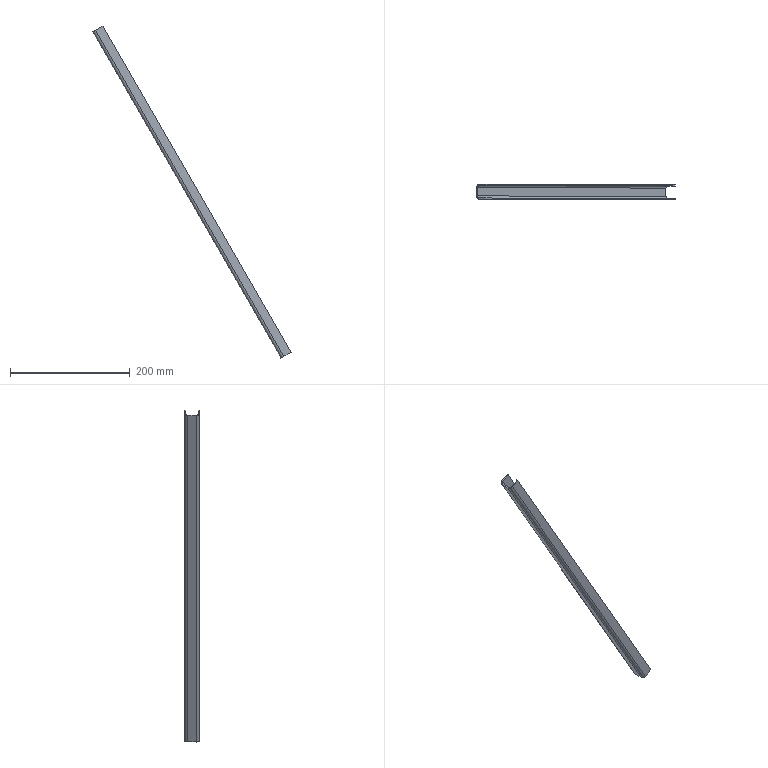Component | SolidWorks | FrontDoorAssembly-1_DoorUpperAndLowerReinforcementBar-2 | 1 solid | 22 faces | box 332.32 x 25 x 555.6 mm | volume 71993 mm3 | plane 18 | cylinder 4 | commonest cylinder face diameters 11 x2 7 x2 | material Malleable Cast Iron
STEP:
#1=COLOUR_RGB('',0.7922,0.8196,0.9333);
#2=FILL_AREA_STYLE_COLOUR('',#1);
#3=FILL_AREA_STYLE('',(#2));
#4=SURFACE_STYLE_FILL_AREA(#3);
#5=SURFACE_SIDE_STYLE('',(#4));
#6=SURFACE_STYLE_USAGE(.BOTH.,#5);
#7=PRESENTATION_STYLE_ASSIGNMENT((#6));
#8=CARTESIAN_POINT('',(10.14,-0.5527,18.399));
#9=VERTEX_POINT('',#8);
#10=CARTESIAN_POINT('',(10.208,-0.5527,18.438));
#11=VERTEX_POINT('',#10);
#12=CARTESIAN_POINT('',(10.14,-0.5527,18.399));
#13=DIRECTION('',(0.866,0.,0.5));
#14=VECTOR('',#13,39.37);
#15=LINE('',#12,#14);
#16=EDGE_CURVE('',#9,#11,#15,.T.);
#17=ORIENTED_EDGE('',*,*,#16,.F.);
#18=CARTESIAN_POINT('',(10.327,-0.3362,18.507));
#19=VERTEX_POINT('',#18);
#20=CARTESIAN_POINT('',(10.327,-0.5527,18.507));
#21=DIRECTION('',(-0.5,-0.,0.866));
#22=DIRECTION('',(0.866,0.,0.5));
#23=AXIS2_PLACEMENT_3D('',#20,#21,#22);
#24=CIRCLE('',#23,0.2165);
#25=EDGE_CURVE('',#19,#9,#24,.T.);
#26=ORIENTED_EDGE('',*,*,#25,.F.);
#27=CARTESIAN_POINT('',(10.327,-0.4149,18.507));
#28=VERTEX_POINT('',#27);
#29=CARTESIAN_POINT('',(10.327,-0.4149,18.507));
#30=DIRECTION('',(-0.,1.,0.));
#31=VECTOR('',#30,39.37);
#32=LINE('',#29,#31);
#33=EDGE_CURVE('',#28,#19,#32,.T.);
#34=ORIENTED_EDGE('',*,*,#33,.F.);
#35=CARTESIAN_POINT('',(10.327,-0.5527,18.507));
#36=DIRECTION('',(-0.5,-0.,0.866));
#37=DIRECTION('',(0.,-1.,0.));
#38=AXIS2_PLACEMENT_3D('',#35,#36,#37);
#39=CIRCLE('',#38,0.1378);
#40=EDGE_CURVE('',#28,#11,#39,.T.);
#41=ORIENTED_EDGE('',*,*,#40,.T.);
#42=EDGE_LOOP('',(#17,#26,#34,#41));
#43=FACE_OUTER_BOUND('',#42,.T.);
#44=CARTESIAN_POINT('',(10.14,-0.5527,18.399));
#45=DIRECTION('',(0.5,0.,-0.866));
#46=DIRECTION('',(0.866,0.,0.5));
#47=AXIS2_PLACEMENT_3D('',#44,#45,#46);
#48=PLANE('',#47);
#49=ADVANCED_FACE('',(#43),#48,.T.);
#50=CARTESIAN_POINT('',(10.14,-1.104,18.399));
#51=VERTEX_POINT('',#50);
#52=CARTESIAN_POINT('',(10.14,-0.3362,18.399));
#53=DIRECTION('',(0.,-1.,-0.));
#54=VECTOR('',#53,39.37);
#55=LINE('',#52,#54);
#56=EDGE_CURVE('',#9,#51,#55,.T.);
#57=ORIENTED_EDGE('',*,*,#56,.F.);
#58=ORIENTED_EDGE('',*,*,#16,.T.);
#59=CARTESIAN_POINT('',(10.208,-1.104,18.438));
#60=VERTEX_POINT('',#59);
#61=CARTESIAN_POINT('',(10.208,-0.3362,18.438));
#62=DIRECTION('',(0.,-1.,-0.));
#63=VECTOR('',#62,39.37);
#64=LINE('',#61,#63);
#65=EDGE_CURVE('',#11,#60,#64,.T.);
#66=ORIENTED_EDGE('',*,*,#65,.T.);
#67=CARTESIAN_POINT('',(10.208,-1.104,18.438));
#68=DIRECTION('',(-0.866,-0.,-0.5));
#69=VECTOR('',#68,39.37);
#70=LINE('',#67,#69);
#71=EDGE_CURVE('',#60,#51,#70,.T.);
#72=ORIENTED_EDGE('',*,*,#71,.T.);
#73=EDGE_LOOP('',(#57,#58,#66,#72));
#74=FACE_OUTER_BOUND('',#73,.T.);
#75=CARTESIAN_POINT('',(10.327,-0.4149,18.507));
#76=DIRECTION('',(0.5,0.,-0.866));
#77=DIRECTION('',(0.866,0.,0.5));
#78=AXIS2_PLACEMENT_3D('',#75,#76,#77);
#79=PLANE('',#78);
#80=ADVANCED_FACE('',(#74),#79,.T.);
#81=CARTESIAN_POINT('',(-2.074,-0.3362,39.987));
#82=VERTEX_POINT('',#81);
#83=CARTESIAN_POINT('',(-2.074,-0.4149,39.987));
#84=VERTEX_POINT('',#83);
#85=CARTESIAN_POINT('',(-2.074,-0.3362,39.987));
#86=DIRECTION('',(0.,-1.,-0.));
#87=VECTOR('',#86,39.37);
#88=LINE('',#85,#87);
#89=EDGE_CURVE('',#82,#84,#88,.T.);
#90=ORIENTED_EDGE('',*,*,#89,.F.);
#91=CARTESIAN_POINT('',(-2.262,-0.5527,39.879));
#92=VERTEX_POINT('',#91);
#93=CARTESIAN_POINT('',(-2.074,-0.5527,39.987));
#94=DIRECTION('',(-0.5,-0.,0.866));
#95=DIRECTION('',(0.866,-0.,0.5));
#96=AXIS2_PLACEMENT_3D('',#93,#94,#95);
#97=CIRCLE('',#96,0.2165);
#98=EDGE_CURVE('',#82,#92,#97,.T.);
#99=ORIENTED_EDGE('',*,*,#98,.T.);
#100=CARTESIAN_POINT('',(-2.193,-0.5527,39.918));
#101=VERTEX_POINT('',#100);
#102=CARTESIAN_POINT('',(-2.193,-0.5527,39.918));
#103=DIRECTION('',(-0.866,-0.,-0.5));
#104=VECTOR('',#103,39.37);
#105=LINE('',#102,#104);
#106=EDGE_CURVE('',#101,#92,#105,.T.);
#107=ORIENTED_EDGE('',*,*,#106,.F.);
#108=CARTESIAN_POINT('',(-2.074,-0.5527,39.987));
#109=DIRECTION('',(-0.5,-0.,0.866));
#110=DIRECTION('',(-0.,-1.,-0.));
#111=AXIS2_PLACEMENT_3D('',#108,#109,#110);
#112=CIRCLE('',#111,0.1378);
#113=EDGE_CURVE('',#84,#101,#112,.T.);
#114=ORIENTED_EDGE('',*,*,#113,.F.);
#115=EDGE_LOOP('',(#90,#99,#107,#114));
#116=FACE_OUTER_BOUND('',#115,.T.);
#117=CARTESIAN_POINT('',(-2.074,-0.3362,39.987));
#118=DIRECTION('',(-0.5,-0.,0.866));
#119=DIRECTION('',(-0.866,-0.,-0.5));
#120=AXIS2_PLACEMENT_3D('',#117,#118,#119);
#121=PLANE('',#120);
#122=ADVANCED_FACE('',(#116),#121,.T.);
#123=CARTESIAN_POINT('',(-1.58,-0.3362,40.273));
#124=VERTEX_POINT('',#123);
#125=CARTESIAN_POINT('',(-1.58,-0.3362,40.273));
#126=DIRECTION('',(-0.866,-0.,-0.5));
#127=VECTOR('',#126,39.37);
#128=LINE('',#125,#127);
#129=EDGE_CURVE('',#124,#82,#128,.T.);
#130=ORIENTED_EDGE('',*,*,#129,.T.);
#131=ORIENTED_EDGE('',*,*,#89,.T.);
#132=CARTESIAN_POINT('',(-1.58,-0.4149,40.273));
#133=VERTEX_POINT('',#132);
#134=CARTESIAN_POINT('',(-1.58,-0.4149,40.273));
#135=DIRECTION('',(-0.866,-0.,-0.5));
#136=VECTOR('',#135,39.37);
#137=LINE('',#134,#136);
#138=EDGE_CURVE('',#133,#84,#137,.T.);
#139=ORIENTED_EDGE('',*,*,#138,.F.);
#140=CARTESIAN_POINT('',(-1.58,-0.4149,40.273));
#141=DIRECTION('',(-0.,1.,0.));
#142=VECTOR('',#141,39.37);
#143=LINE('',#140,#142);
#144=EDGE_CURVE('',#133,#124,#143,.T.);
#145=ORIENTED_EDGE('',*,*,#144,.T.);
#146=EDGE_LOOP('',(#130,#131,#139,#145));
#147=FACE_OUTER_BOUND('',#146,.T.);
#148=CARTESIAN_POINT('',(-2.193,-0.5527,39.918));
#149=DIRECTION('',(-0.5,-0.,0.866));
#150=DIRECTION('',(-0.866,-0.,-0.5));
#151=AXIS2_PLACEMENT_3D('',#148,#149,#150);
#152=PLANE('',#151);
#153=ADVANCED_FACE('',(#147),#152,.T.);
#154=CARTESIAN_POINT('',(10.327,-1.32,18.507));
#155=VERTEX_POINT('',#154);
#156=CARTESIAN_POINT('',(10.327,-1.242,18.507));
#157=VERTEX_POINT('',#156);
#158=CARTESIAN_POINT('',(10.327,-1.32,18.507));
#159=DIRECTION('',(-0.,1.,0.));
#160=VECTOR('',#159,39.37);
#161=LINE('',#158,#160);
#162=EDGE_CURVE('',#155,#157,#161,.T.);
#163=ORIENTED_EDGE('',*,*,#162,.F.);
#164=CARTESIAN_POINT('',(10.327,-1.104,18.507));
#165=DIRECTION('',(-0.5,-0.,0.866));
#166=DIRECTION('',(0.866,0.,0.5));
#167=AXIS2_PLACEMENT_3D('',#164,#165,#166);
#168=CIRCLE('',#167,0.2165);
#169=EDGE_CURVE('',#51,#155,#168,.T.);
#170=ORIENTED_EDGE('',*,*,#169,.F.);
#171=ORIENTED_EDGE('',*,*,#71,.F.);
#172=CARTESIAN_POINT('',(10.327,-1.104,18.507));
#173=DIRECTION('',(-0.5,-0.,0.866));
#174=DIRECTION('',(-0.,-1.,-0.));
#175=AXIS2_PLACEMENT_3D('',#172,#173,#174);
#176=CIRCLE('',#175,0.1378);
#177=EDGE_CURVE('',#60,#157,#176,.T.);
#178=ORIENTED_EDGE('',*,*,#177,.T.);
#179=EDGE_LOOP('',(#163,#170,#171,#178));
#180=FACE_OUTER_BOUND('',#179,.T.);
#181=CARTESIAN_POINT('',(10.327,-1.32,18.507));
#182=DIRECTION('',(0.5,0.,-0.866));
#183=DIRECTION('',(0.866,0.,0.5));
#184=AXIS2_PLACEMENT_3D('',#181,#182,#183);
#185=PLANE('',#184);
#186=ADVANCED_FACE('',(#180),#185,.T.);
#187=CARTESIAN_POINT('',(10.822,-1.32,18.793));
#188=VERTEX_POINT('',#187);
#189=CARTESIAN_POINT('',(10.14,-1.32,18.399));
#190=DIRECTION('',(0.866,0.,0.5));
#191=VECTOR('',#190,39.37);
#192=LINE('',#189,#191);
#193=EDGE_CURVE('',#155,#188,#192,.T.);
#194=ORIENTED_EDGE('',*,*,#193,.F.);
#195=ORIENTED_EDGE('',*,*,#162,.T.);
#196=CARTESIAN_POINT('',(10.822,-1.242,18.793));
#197=VERTEX_POINT('',#196);
#198=CARTESIAN_POINT('',(10.14,-1.242,18.399));
#199=DIRECTION('',(0.866,0.,0.5));
#200=VECTOR('',#199,39.37);
#201=LINE('',#198,#200);
#202=EDGE_CURVE('',#157,#197,#201,.T.);
#203=ORIENTED_EDGE('',*,*,#202,.T.);
#204=CARTESIAN_POINT('',(10.822,-1.32,18.793));
#205=DIRECTION('',(-0.,1.,0.));
#206=VECTOR('',#205,39.37);
#207=LINE('',#204,#206);
#208=EDGE_CURVE('',#188,#197,#207,.T.);
#209=ORIENTED_EDGE('',*,*,#208,.F.);
#210=EDGE_LOOP('',(#194,#195,#203,#209));
#211=FACE_OUTER_BOUND('',#210,.T.);
#212=CARTESIAN_POINT('',(10.208,-1.104,18.438));
#213=DIRECTION('',(0.5,0.,-0.866));
#214=DIRECTION('',(0.866,0.,0.5));
#215=AXIS2_PLACEMENT_3D('',#212,#213,#214);
#216=PLANE('',#215);
#217=ADVANCED_FACE('',(#211),#216,.T.);
#218=CARTESIAN_POINT('',(-2.262,-1.104,39.879));
#219=VERTEX_POINT('',#218);
#220=CARTESIAN_POINT('',(-2.193,-1.104,39.918));
#221=VERTEX_POINT('',#220);
#222=CARTESIAN_POINT('',(-2.262,-1.104,39.879));
#223=DIRECTION('',(0.866,0.,0.5));
#224=VECTOR('',#223,39.37);
#225=LINE('',#222,#224);
#226=EDGE_CURVE('',#219,#221,#225,.T.);
#227=ORIENTED_EDGE('',*,*,#226,.F.);
#228=CARTESIAN_POINT('',(-2.074,-1.32,39.987));
#229=VERTEX_POINT('',#228);
#230=CARTESIAN_POINT('',(-2.074,-1.104,39.987));
#231=DIRECTION('',(-0.5,-0.,0.866));
#232=DIRECTION('',(0.866,-0.,0.5));
#233=AXIS2_PLACEMENT_3D('',#230,#231,#232);
#234=CIRCLE('',#233,0.2165);
#235=EDGE_CURVE('',#219,#229,#234,.T.);
#236=ORIENTED_EDGE('',*,*,#235,.T.);
#237=CARTESIAN_POINT('',(-2.074,-1.242,39.987));
#238=VERTEX_POINT('',#237);
#239=CARTESIAN_POINT('',(-2.074,-1.242,39.987));
#240=DIRECTION('',(0.,-1.,-0.));
#241=VECTOR('',#240,39.37);
#242=LINE('',#239,#241);
#243=EDGE_CURVE('',#238,#229,#242,.T.);
#244=ORIENTED_EDGE('',*,*,#243,.F.);
#245=CARTESIAN_POINT('',(-2.074,-1.104,39.987));
#246=DIRECTION('',(-0.5,-0.,0.866));
#247=DIRECTION('',(-0.,-1.,0.));
#248=AXIS2_PLACEMENT_3D('',#245,#246,#247);
#249=CIRCLE('',#248,0.1378);
#250=EDGE_CURVE('',#221,#238,#249,.T.);
#251=ORIENTED_EDGE('',*,*,#250,.F.);
#252=EDGE_LOOP('',(#227,#236,#244,#251));
#253=FACE_OUTER_BOUND('',#252,.T.);
#254=CARTESIAN_POINT('',(-2.262,-1.104,39.879));
#255=DIRECTION('',(-0.5,-0.,0.866));
#256=DIRECTION('',(-0.866,-0.,-0.5));
#257=AXIS2_PLACEMENT_3D('',#254,#255,#256);
#258=PLANE('',#257);
#259=ADVANCED_FACE('',(#253),#258,.T.);
#260=CARTESIAN_POINT('',(-2.262,-0.3362,39.879));
#261=DIRECTION('',(0.,-1.,-0.));
#262=VECTOR('',#261,39.37);
#263=LINE('',#260,#262);
#264=EDGE_CURVE('',#92,#219,#263,.T.);
#265=ORIENTED_EDGE('',*,*,#264,.T.);
#266=ORIENTED_EDGE('',*,*,#226,.T.);
#267=CARTESIAN_POINT('',(-2.193,-0.3362,39.918));
#268=DIRECTION('',(0.,-1.,-0.));
#269=VECTOR('',#268,39.37);
#270=LINE('',#267,#269);
#271=EDGE_CURVE('',#101,#221,#270,.T.);
#272=ORIENTED_EDGE('',*,*,#271,.F.);
#273=ORIENTED_EDGE('',*,*,#106,.T.);
#274=EDGE_LOOP('',(#265,#266,#272,#273));
#275=FACE_OUTER_BOUND('',#274,.T.);
#276=CARTESIAN_POINT('',(-2.074,-1.242,39.987));
#277=DIRECTION('',(-0.5,-0.,0.866));
#278=DIRECTION('',(-0.866,-0.,-0.5));
#279=AXIS2_PLACEMENT_3D('',#276,#277,#278);
#280=PLANE('',#279);
#281=ADVANCED_FACE('',(#275),#280,.T.);
#282=CARTESIAN_POINT('',(-1.58,-1.242,40.273));
#283=VERTEX_POINT('',#282);
#284=CARTESIAN_POINT('',(-2.262,-1.242,39.879));
#285=DIRECTION('',(0.866,0.,0.5));
#286=VECTOR('',#285,39.37);
#287=LINE('',#284,#286);
#288=EDGE_CURVE('',#238,#283,#287,.T.);
#289=ORIENTED_EDGE('',*,*,#288,.T.);
#290=CARTESIAN_POINT('',(10.822,-1.242,18.793));
#291=DIRECTION('',(-0.5,-0.,0.866));
#292=VECTOR('',#291,39.37);
#293=LINE('',#290,#292);
#294=EDGE_CURVE('',#197,#283,#293,.T.);
#295=ORIENTED_EDGE('',*,*,#294,.F.);
#296=ORIENTED_EDGE('',*,*,#202,.F.);
#297=CARTESIAN_POINT('',(10.327,-1.242,18.507));
#298=DIRECTION('',(-0.5,-0.,0.866));
#299=VECTOR('',#298,39.37);
#300=LINE('',#297,#299);
#301=EDGE_CURVE('',#157,#238,#300,.T.);
#302=ORIENTED_EDGE('',*,*,#301,.T.);
#303=EDGE_LOOP('',(#289,#295,#296,#302));
#304=FACE_OUTER_BOUND('',#303,.T.);
#305=CARTESIAN_POINT('',(10.14,-1.242,18.399));
#306=DIRECTION('',(0.,-1.,-0.));
#307=DIRECTION('',(-0.866,-0.,-0.5));
#308=AXIS2_PLACEMENT_3D('',#305,#306,#307);
#309=PLANE('',#308);
#310=ADVANCED_FACE('',(#304),#309,.F.);
#311=CARTESIAN_POINT('',(-1.58,-1.32,40.273));
#312=VERTEX_POINT('',#311);
#313=CARTESIAN_POINT('',(-1.58,-1.32,40.273));
#314=DIRECTION('',(-0.,1.,0.));
#315=VECTOR('',#314,39.37);
#316=LINE('',#313,#315);
#317=EDGE_CURVE('',#312,#283,#316,.T.);
#318=ORIENTED_EDGE('',*,*,#317,.F.);
#319=CARTESIAN_POINT('',(10.822,-1.32,18.793));
#320=DIRECTION('',(-0.5,-0.,0.866));
#321=VECTOR('',#320,39.37);
#322=LINE('',#319,#321);
#323=EDGE_CURVE('',#188,#312,#322,.T.);
#324=ORIENTED_EDGE('',*,*,#323,.F.);
#325=ORIENTED_EDGE('',*,*,#208,.T.);
#326=ORIENTED_EDGE('',*,*,#294,.T.);
#327=EDGE_LOOP('',(#318,#324,#325,#326));
#328=FACE_OUTER_BOUND('',#327,.T.);
#329=CARTESIAN_POINT('',(10.822,-1.32,18.793));
#330=DIRECTION('',(0.866,0.,0.5));
#331=DIRECTION('',(0.,-1.,-0.));
#332=AXIS2_PLACEMENT_3D('',#329,#330,#331);
#333=PLANE('',#332);
#334=ADVANCED_FACE('',(#328),#333,.T.);
#335=CARTESIAN_POINT('',(-2.262,-1.32,39.879));
#336=DIRECTION('',(0.866,0.,0.5));
#337=VECTOR('',#336,39.37);
#338=LINE('',#335,#337);
#339=EDGE_CURVE('',#229,#312,#338,.T.);
#340=ORIENTED_EDGE('',*,*,#339,.F.);
#341=CARTESIAN_POINT('',(10.327,-1.32,18.507));
#342=DIRECTION('',(-0.5,-0.,0.866));
#343=VECTOR('',#342,39.37);
#344=LINE('',#341,#343);
#345=EDGE_CURVE('',#155,#229,#344,.T.);
#346=ORIENTED_EDGE('',*,*,#345,.F.);
#347=ORIENTED_EDGE('',*,*,#193,.T.);
#348=ORIENTED_EDGE('',*,*,#323,.T.);
#349=EDGE_LOOP('',(#340,#346,#347,#348));
#350=FACE_OUTER_BOUND('',#349,.T.);
#351=CARTESIAN_POINT('',(10.14,-1.32,18.399));
#352=DIRECTION('',(0.,-1.,-0.));
#353=DIRECTION('',(-0.866,-0.,-0.5));
#354=AXIS2_PLACEMENT_3D('',#351,#352,#353);
#355=PLANE('',#354);
#356=ADVANCED_FACE('',(#350),#355,.T.);
#357=ORIENTED_EDGE('',*,*,#235,.F.);
#358=CARTESIAN_POINT('',(10.14,-1.104,18.399));
#359=DIRECTION('',(-0.5,-0.,0.866));
#360=VECTOR('',#359,39.37);
#361=LINE('',#358,#360);
#362=EDGE_CURVE('',#51,#219,#361,.T.);
#363=ORIENTED_EDGE('',*,*,#362,.F.);
#364=ORIENTED_EDGE('',*,*,#169,.T.);
#365=ORIENTED_EDGE('',*,*,#345,.T.);
#366=EDGE_LOOP('',(#357,#363,#364,#365));
#367=FACE_OUTER_BOUND('',#366,.T.);
#368=CARTESIAN_POINT('',(10.327,-1.104,18.507));
#369=DIRECTION('',(-0.5,-0.,0.866));
#370=DIRECTION('',(-0.866,-0.,-0.5));
#371=AXIS2_PLACEMENT_3D('',#368,#369,#370);
#372=CYLINDRICAL_SURFACE('',#371,0.2165);
#373=ADVANCED_FACE('',(#367),#372,.T.);
#374=ORIENTED_EDGE('',*,*,#264,.F.);
#375=CARTESIAN_POINT('',(10.14,-0.5527,18.399));
#376=DIRECTION('',(-0.5,-0.,0.866));
#377=VECTOR('',#376,39.37);
#378=LINE('',#375,#377);
#379=EDGE_CURVE('',#9,#92,#378,.T.);
#380=ORIENTED_EDGE('',*,*,#379,.F.);
#381=ORIENTED_EDGE('',*,*,#56,.T.);
#382=ORIENTED_EDGE('',*,*,#362,.T.);
#383=EDGE_LOOP('',(#374,#380,#381,#382));
#384=FACE_OUTER_BOUND('',#383,.T.);
#385=CARTESIAN_POINT('',(10.14,-0.3362,18.399));
#386=DIRECTION('',(-0.866,-0.,-0.5));
#387=DIRECTION('',(-0.,1.,0.));
#388=AXIS2_PLACEMENT_3D('',#385,#386,#387);
#389=PLANE('',#388);
#390=ADVANCED_FACE('',(#384),#389,.T.);
#391=ORIENTED_EDGE('',*,*,#98,.F.);
#392=CARTESIAN_POINT('',(10.327,-0.3362,18.507));
#393=DIRECTION('',(-0.5,-0.,0.866));
#394=VECTOR('',#393,39.37);
#395=LINE('',#392,#394);
#396=EDGE_CURVE('',#19,#82,#395,.T.);
#397=ORIENTED_EDGE('',*,*,#396,.F.);
#398=ORIENTED_EDGE('',*,*,#25,.T.);
#399=ORIENTED_EDGE('',*,*,#379,.T.);
#400=EDGE_LOOP('',(#391,#397,#398,#399));
#401=FACE_OUTER_BOUND('',#400,.T.);
#402=CARTESIAN_POINT('',(10.327,-0.5527,18.507));
#403=DIRECTION('',(-0.5,-0.,0.866));
#404=DIRECTION('',(-0.866,-0.,-0.5));
#405=AXIS2_PLACEMENT_3D('',#402,#403,#404);
#406=CYLINDRICAL_SURFACE('',#405,0.2165);
#407=ADVANCED_FACE('',(#401),#406,.T.);
#408=ORIENTED_EDGE('',*,*,#129,.F.);
#409=CARTESIAN_POINT('',(10.822,-0.3362,18.793));
#410=VERTEX_POINT('',#409);
#411=CARTESIAN_POINT('',(10.822,-0.3362,18.793));
#412=DIRECTION('',(-0.5,-0.,0.866));
#413=VECTOR('',#412,39.37);
#414=LINE('',#411,#413);
#415=EDGE_CURVE('',#410,#124,#414,.T.);
#416=ORIENTED_EDGE('',*,*,#415,.F.);
#417=CARTESIAN_POINT('',(10.822,-0.3362,18.793));
#418=DIRECTION('',(-0.866,-0.,-0.5));
#419=VECTOR('',#418,39.37);
#420=LINE('',#417,#419);
#421=EDGE_CURVE('',#410,#19,#420,.T.);
#422=ORIENTED_EDGE('',*,*,#421,.T.);
#423=ORIENTED_EDGE('',*,*,#396,.T.);
#424=EDGE_LOOP('',(#408,#416,#422,#423));
#425=FACE_OUTER_BOUND('',#424,.T.);
#426=CARTESIAN_POINT('',(10.822,-0.3362,18.793));
#427=DIRECTION('',(-0.,1.,0.));
#428=DIRECTION('',(0.866,0.,0.5));
#429=AXIS2_PLACEMENT_3D('',#426,#427,#428);
#430=PLANE('',#429);
#431=ADVANCED_FACE('',(#425),#430,.T.);
#432=ORIENTED_EDGE('',*,*,#144,.F.);
#433=CARTESIAN_POINT('',(10.822,-0.4149,18.793));
#434=VERTEX_POINT('',#433);
#435=CARTESIAN_POINT('',(10.822,-0.4149,18.793));
#436=DIRECTION('',(-0.5,-0.,0.866));
#437=VECTOR('',#436,39.37);
#438=LINE('',#435,#437);
#439=EDGE_CURVE('',#434,#133,#438,.T.);
#440=ORIENTED_EDGE('',*,*,#439,.F.);
#441=CARTESIAN_POINT('',(10.822,-0.4149,18.793));
#442=DIRECTION('',(-0.,1.,0.));
#443=VECTOR('',#442,39.37);
#444=LINE('',#441,#443);
#445=EDGE_CURVE('',#434,#410,#444,.T.);
#446=ORIENTED_EDGE('',*,*,#445,.T.);
#447=ORIENTED_EDGE('',*,*,#415,.T.);
#448=EDGE_LOOP('',(#432,#440,#446,#447));
#449=FACE_OUTER_BOUND('',#448,.T.);
#450=CARTESIAN_POINT('',(10.822,-0.4149,18.793));
#451=DIRECTION('',(0.866,0.,0.5));
#452=DIRECTION('',(0.,-1.,-0.));
#453=AXIS2_PLACEMENT_3D('',#450,#451,#452);
#454=PLANE('',#453);
#455=ADVANCED_FACE('',(#449),#454,.T.);
#456=ORIENTED_EDGE('',*,*,#138,.T.);
#457=CARTESIAN_POINT('',(10.327,-0.4149,18.507));
#458=DIRECTION('',(-0.5,-0.,0.866));
#459=VECTOR('',#458,39.37);
#460=LINE('',#457,#459);
#461=EDGE_CURVE('',#28,#84,#460,.T.);
#462=ORIENTED_EDGE('',*,*,#461,.F.);
#463=CARTESIAN_POINT('',(10.822,-0.4149,18.793));
#464=DIRECTION('',(-0.866,-0.,-0.5));
#465=VECTOR('',#464,39.37);
#466=LINE('',#463,#465);
#467=EDGE_CURVE('',#434,#28,#466,.T.);
#468=ORIENTED_EDGE('',*,*,#467,.F.);
#469=ORIENTED_EDGE('',*,*,#439,.T.);
#470=EDGE_LOOP('',(#456,#462,#468,#469));
#471=FACE_OUTER_BOUND('',#470,.T.);
#472=CARTESIAN_POINT('',(10.822,-0.4149,18.793));
#473=DIRECTION('',(-0.,1.,0.));
#474=DIRECTION('',(0.866,0.,0.5));
#475=AXIS2_PLACEMENT_3D('',#472,#473,#474);
#476=PLANE('',#475);
#477=ADVANCED_FACE('',(#471),#476,.F.);
#478=ORIENTED_EDGE('',*,*,#113,.T.);
#479=CARTESIAN_POINT('',(10.208,-0.5527,18.438));
#480=DIRECTION('',(-0.5,-0.,0.866));
#481=VECTOR('',#480,39.37);
#482=LINE('',#479,#481);
#483=EDGE_CURVE('',#11,#101,#482,.T.);
#484=ORIENTED_EDGE('',*,*,#483,.F.);
#485=ORIENTED_EDGE('',*,*,#40,.F.);
#486=ORIENTED_EDGE('',*,*,#461,.T.);
#487=EDGE_LOOP('',(#478,#484,#485,#486));
#488=FACE_OUTER_BOUND('',#487,.T.);
#489=CARTESIAN_POINT('',(10.327,-0.5527,18.507));
#490=DIRECTION('',(-0.5,-0.,0.866));
#491=DIRECTION('',(-0.866,-0.,-0.5));
#492=AXIS2_PLACEMENT_3D('',#489,#490,#491);
#493=CYLINDRICAL_SURFACE('',#492,0.1378);
#494=ADVANCED_FACE('',(#488),#493,.F.);
#495=ORIENTED_EDGE('',*,*,#271,.T.);
#496=CARTESIAN_POINT('',(10.208,-1.104,18.438));
#497=DIRECTION('',(-0.5,-0.,0.866));
#498=VECTOR('',#497,39.37);
#499=LINE('',#496,#498);
#500=EDGE_CURVE('',#60,#221,#499,.T.);
#501=ORIENTED_EDGE('',*,*,#500,.F.);
#502=ORIENTED_EDGE('',*,*,#65,.F.);
#503=ORIENTED_EDGE('',*,*,#483,.T.);
#504=EDGE_LOOP('',(#495,#501,#502,#503));
#505=FACE_OUTER_BOUND('',#504,.T.);
#506=CARTESIAN_POINT('',(10.208,-0.3362,18.438));
#507=DIRECTION('',(-0.866,-0.,-0.5));
#508=DIRECTION('',(-0.,1.,0.));
#509=AXIS2_PLACEMENT_3D('',#506,#507,#508);
#510=PLANE('',#509);
#511=ADVANCED_FACE('',(#505),#510,.F.);
#512=ORIENTED_EDGE('',*,*,#250,.T.);
#513=ORIENTED_EDGE('',*,*,#301,.F.);
#514=ORIENTED_EDGE('',*,*,#177,.F.);
#515=ORIENTED_EDGE('',*,*,#500,.T.);
#516=EDGE_LOOP('',(#512,#513,#514,#515));
#517=FACE_OUTER_BOUND('',#516,.T.);
#518=CARTESIAN_POINT('',(10.327,-1.104,18.507));
#519=DIRECTION('',(-0.5,-0.,0.866));
#520=DIRECTION('',(-0.866,-0.,-0.5));
#521=AXIS2_PLACEMENT_3D('',#518,#519,#520);
#522=CYLINDRICAL_SURFACE('',#521,0.1378);
#523=ADVANCED_FACE('',(#517),#522,.F.);
#524=ORIENTED_EDGE('',*,*,#467,.T.);
#525=ORIENTED_EDGE('',*,*,#33,.T.);
#526=ORIENTED_EDGE('',*,*,#421,.F.);
#527=ORIENTED_EDGE('',*,*,#445,.F.);
#528=EDGE_LOOP('',(#524,#525,#526,#527));
#529=FACE_OUTER_BOUND('',#528,.T.);
#530=CARTESIAN_POINT('',(10.327,-1.104,18.507));
#531=DIRECTION('',(0.5,0.,-0.866));
#532=DIRECTION('',(0.,-1.,-0.));
#533=AXIS2_PLACEMENT_3D('',#530,#531,#532);
#534=PLANE('',#533);
#535=ADVANCED_FACE('',(#529),#534,.T.);
#536=ORIENTED_EDGE('',*,*,#288,.F.);
#537=ORIENTED_EDGE('',*,*,#243,.T.);
#538=ORIENTED_EDGE('',*,*,#339,.T.);
#539=ORIENTED_EDGE('',*,*,#317,.T.);
#540=EDGE_LOOP('',(#536,#537,#538,#539));
#541=FACE_OUTER_BOUND('',#540,.T.);
#542=CARTESIAN_POINT('',(-2.074,-1.104,39.987));
#543=DIRECTION('',(0.5,0.,-0.866));
#544=DIRECTION('',(0.,-1.,-0.));
#545=AXIS2_PLACEMENT_3D('',#542,#543,#544);
#546=PLANE('',#545);
#547=ADVANCED_FACE('',(#541),#546,.F.);
#548=CLOSED_SHELL('',(#49,#80,#122,#153,#186,#217,#259,#281,#310,#334,#356,#373,#390,#407,#431,#455,#477,#494,#511,#523,#535,#547));
#549=MANIFOLD_SOLID_BREP('',#548);
#550=STYLED_ITEM('',(#7),#549);
#551=(LENGTH_UNIT()NAMED_UNIT(*)SI_UNIT($,.METRE.));
#552=LENGTH_MEASURE_WITH_UNIT(LENGTH_MEASURE(0.0254),#551);
#553=DIMENSIONAL_EXPONENTS(1.,0.,0.,0.,0.,0.,0.);
#554=(CONVERSION_BASED_UNIT('',#552)LENGTH_UNIT()NAMED_UNIT(#553));
#555=UNCERTAINTY_MEASURE_WITH_UNIT(LENGTH_MEASURE(0.00001),#554,'','');
#556=(NAMED_UNIT(*)PLANE_ANGLE_UNIT()SI_UNIT($,.RADIAN.));
#557=(NAMED_UNIT(*)SI_UNIT($,.STERADIAN.)SOLID_ANGLE_UNIT());
#558=(GEOMETRIC_REPRESENTATION_CONTEXT(3)GLOBAL_UNCERTAINTY_ASSIGNED_CONTEXT((#555))GLOBAL_UNIT_ASSIGNED_CONTEXT((#554,#556,#557))REPRESENTATION_CONTEXT('',''));
#559=MECHANICAL_DESIGN_GEOMETRIC_PRESENTATION_REPRESENTATION('',(#550),#558);
#560=CARTESIAN_POINT('',(0.,0.,0.));
#561=DIRECTION('',(0.,0.,1.));
#562=DIRECTION('',(1.,0.,0.));
#563=AXIS2_PLACEMENT_3D('',#560,#561,#562);
#564=(LENGTH_UNIT()NAMED_UNIT(*)SI_UNIT($,.METRE.));
#565=LENGTH_MEASURE_WITH_UNIT(LENGTH_MEASURE(0.0254),#564);
#566=DIMENSIONAL_EXPONENTS(1.,0.,0.,0.,0.,0.,0.);
#567=(CONVERSION_BASED_UNIT('',#565)LENGTH_UNIT()NAMED_UNIT(#566));
#568=UNCERTAINTY_MEASURE_WITH_UNIT(LENGTH_MEASURE(0.00001),#567,'','');
#569=(NAMED_UNIT(*)PLANE_ANGLE_UNIT()SI_UNIT($,.RADIAN.));
#570=(NAMED_UNIT(*)SI_UNIT($,.STERADIAN.)SOLID_ANGLE_UNIT());
#571=(GEOMETRIC_REPRESENTATION_CONTEXT(3)GLOBAL_UNCERTAINTY_ASSIGNED_CONTEXT((#568))GLOBAL_UNIT_ASSIGNED_CONTEXT((#567,#569,#570))REPRESENTATION_CONTEXT('',''));
#572=ADVANCED_BREP_SHAPE_REPRESENTATION('',(#549,#563),#571);
#573=PRESENTATION_LAYER_ASSIGNMENT('','',(#550));